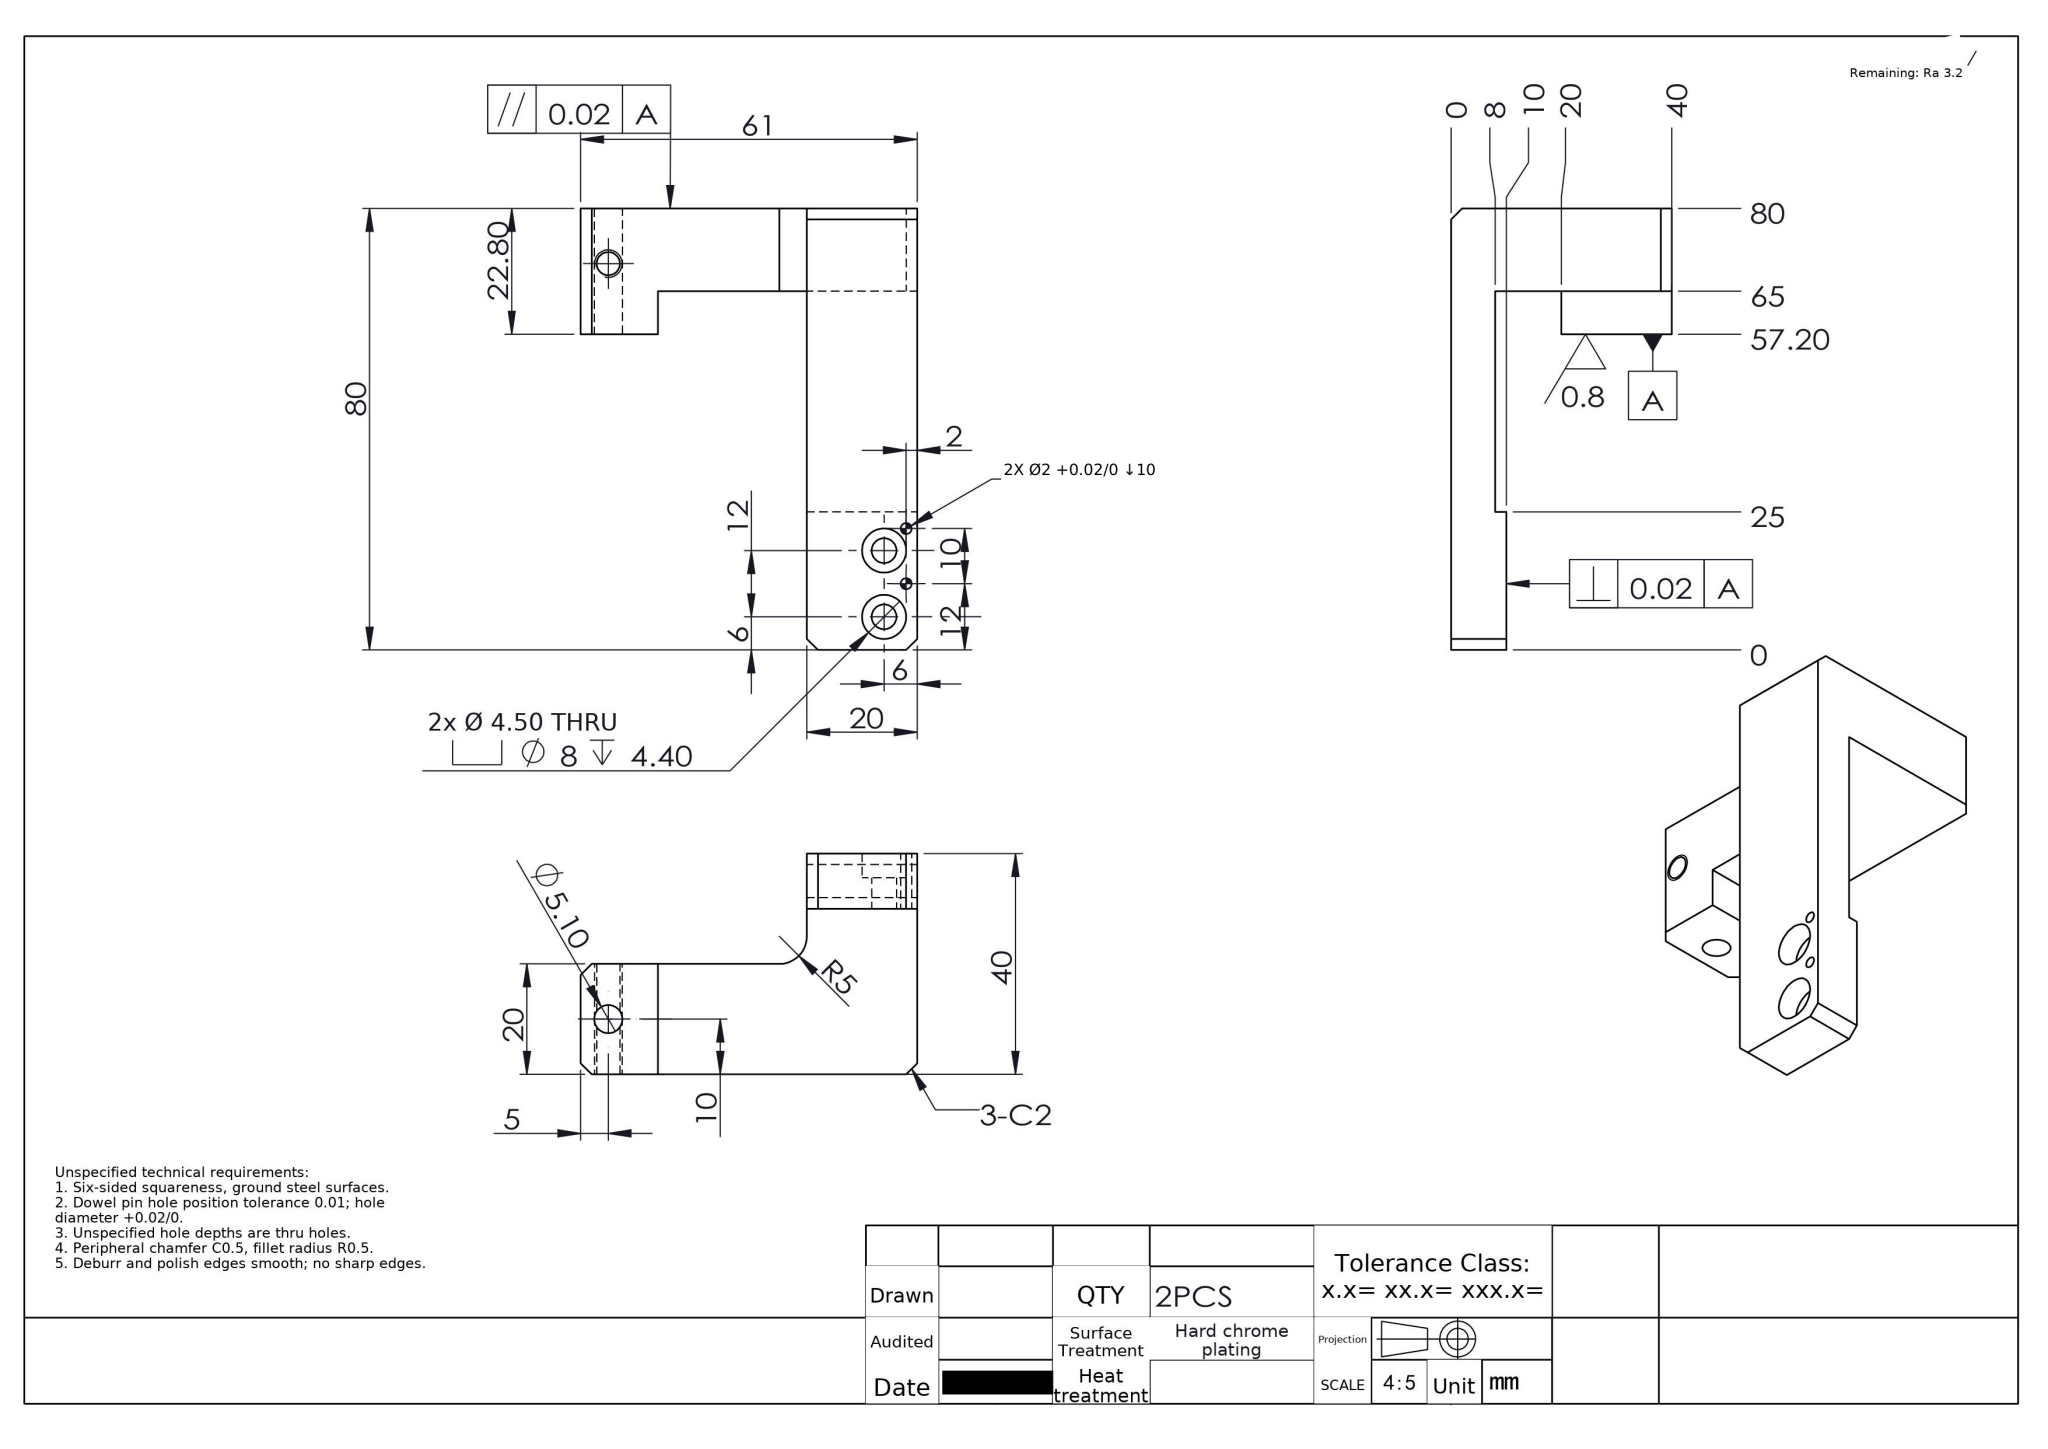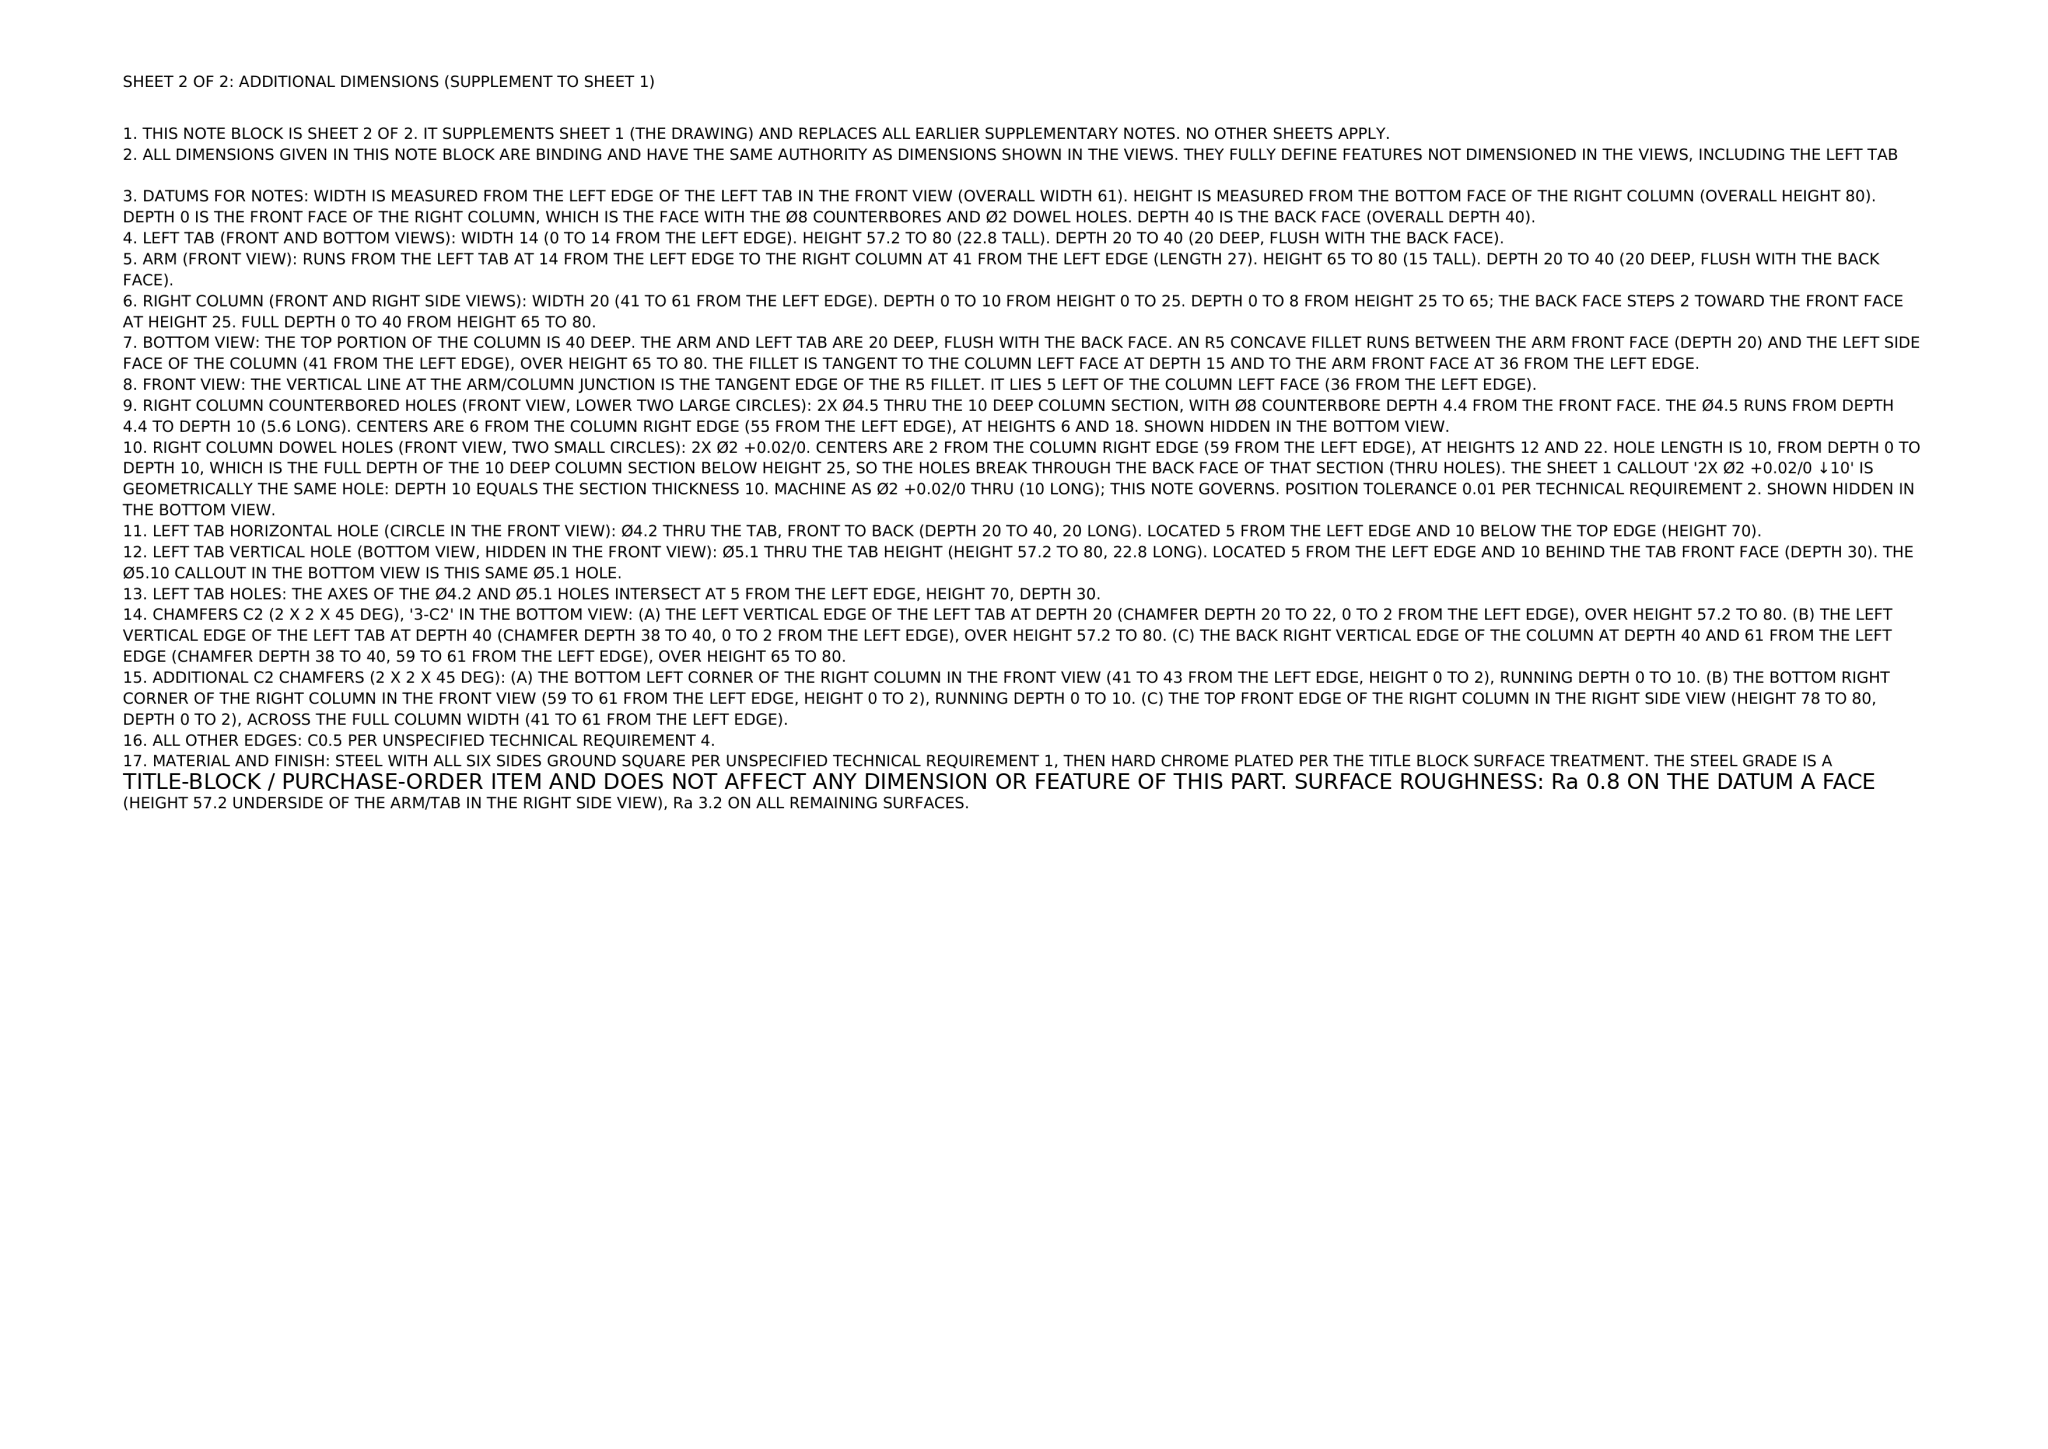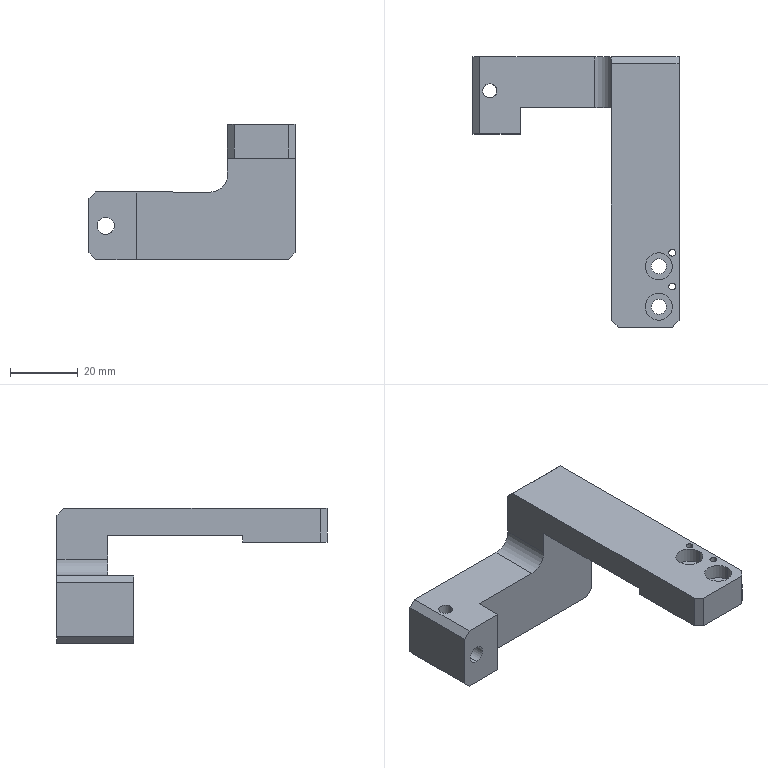Part | NX | mm | 1 solid | 41 faces | box 61 x 80 x 40 mm | volume 36401 mm3 | plane 22 | cylinder 19 | commonest cylinder face diameters 4.2 x4 2 x4 8 x4 4.5 x4 5.1 x2 10 x1